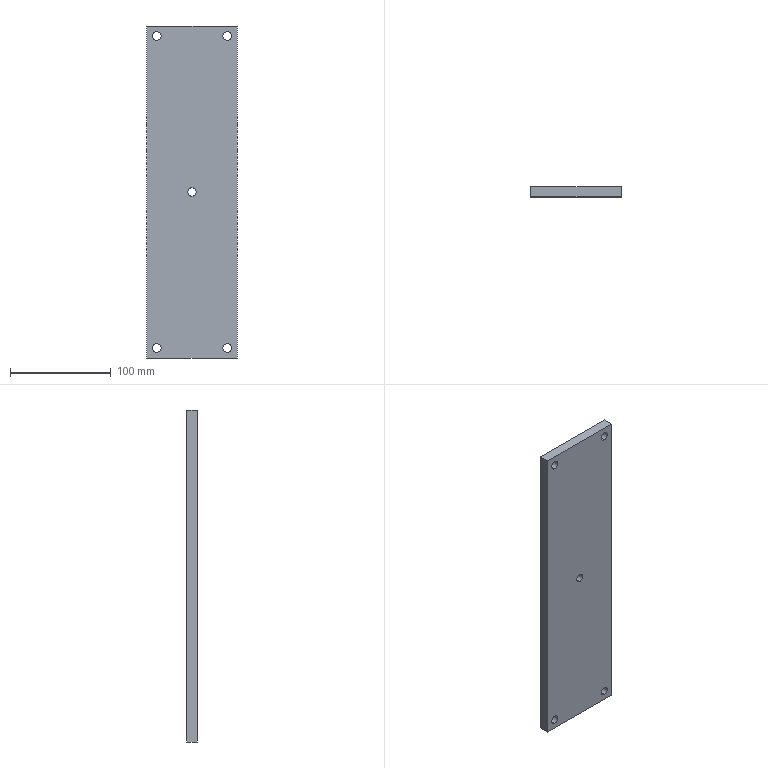Component | SolidWorks | SL021-102-4100.SL4PRT-1 | 1 solid | 16 faces | box 90 x 10 x 330 mm | volume 294163 mm3 | cylinder 10 | plane 6 | commonest cylinder face diameters 8.5 x10 | material AL6061
build123d program:
from build123d import *

# Parameters (mm, degrees)
SKETCH1_W                  = 330
SKETCH1_H                  = 90
BOSS_EXTRUDE1_DEPTH        = 5
F_8_5_8_5_DIAMETER_HOLE1_D = 8.5


with BuildPart() as part:
    # Sketch1 → Boss-Extrude1 (new, symmetric)
    with BuildSketch(Plane.XY):
        Rectangle(SKETCH1_W, SKETCH1_H)
    extrude(amount=BOSS_EXTRUDE1_DEPTH, both=True)

    # 8.5 _8.5_ Diameter Hole1 (through all)
    with Locations(Plane.XY.offset(5)):
        with Locations((-155, 35), (-155, -35), (155, -35), (155, 35), (0, 0)):
            Hole(F_8_5_8_5_DIAMETER_HOLE1_D / 2)


solid = part.part

# Placed as in the assembly
solid = solid.moved(Location((-91.163, 64.501, -151.378), (90, 0, 90)))
STEP:
#1=COLOUR_RGB('',0.7922,0.8196,0.9333);
#2=FILL_AREA_STYLE_COLOUR('',#1);
#3=FILL_AREA_STYLE('',(#2));
#4=SURFACE_STYLE_FILL_AREA(#3);
#5=SURFACE_SIDE_STYLE('',(#4));
#6=SURFACE_STYLE_USAGE(.BOTH.,#5);
#7=PRESENTATION_STYLE_ASSIGNMENT((#6));
#8=CARTESIAN_POINT('',(-4.967,2.736,-12.229));
#9=VERTEX_POINT('',#8);
#10=CARTESIAN_POINT('',(-4.967,2.736,-11.895));
#11=VERTEX_POINT('',#10);
#12=CARTESIAN_POINT('',(-4.967,2.736,-12.062));
#13=DIRECTION('',(0.,-1.,0.));
#14=DIRECTION('',(0.,0.,1.));
#15=AXIS2_PLACEMENT_3D('',#12,#13,#14);
#16=CIRCLE('',#15,0.1673);
#17=EDGE_CURVE('',#9,#11,#16,.T.);
#18=ORIENTED_EDGE('',*,*,#17,.F.);
#19=CARTESIAN_POINT('',(-4.967,2.343,-12.229));
#20=VERTEX_POINT('',#19);
#21=CARTESIAN_POINT('',(-4.967,2.343,-12.229));
#22=DIRECTION('',(0.,-1.,0.));
#23=VECTOR('',#22,39.37);
#24=LINE('',#21,#23);
#25=EDGE_CURVE('',#9,#20,#24,.T.);
#26=ORIENTED_EDGE('',*,*,#25,.T.);
#27=CARTESIAN_POINT('',(-4.967,2.343,-11.895));
#28=VERTEX_POINT('',#27);
#29=CARTESIAN_POINT('',(-4.967,2.343,-12.062));
#30=DIRECTION('',(0.,-1.,0.));
#31=DIRECTION('',(0.,0.,1.));
#32=AXIS2_PLACEMENT_3D('',#29,#30,#31);
#33=CIRCLE('',#32,0.1673);
#34=EDGE_CURVE('',#20,#28,#33,.T.);
#35=ORIENTED_EDGE('',*,*,#34,.T.);
#36=CARTESIAN_POINT('',(-4.967,2.343,-11.895));
#37=DIRECTION('',(0.,-1.,0.));
#38=VECTOR('',#37,39.37);
#39=LINE('',#36,#38);
#40=EDGE_CURVE('',#11,#28,#39,.T.);
#41=ORIENTED_EDGE('',*,*,#40,.F.);
#42=EDGE_LOOP('',(#18,#26,#35,#41));
#43=FACE_OUTER_BOUND('',#42,.T.);
#44=CARTESIAN_POINT('',(-4.967,2.343,-12.062));
#45=DIRECTION('',(0.,-1.,0.));
#46=DIRECTION('',(0.,0.,1.));
#47=AXIS2_PLACEMENT_3D('',#44,#45,#46);
#48=CYLINDRICAL_SURFACE('',#47,0.1673);
#49=ADVANCED_FACE('',(#43),#48,.F.);
#50=CARTESIAN_POINT('',(-2.211,2.736,-12.229));
#51=VERTEX_POINT('',#50);
#52=CARTESIAN_POINT('',(-2.211,2.736,-11.895));
#53=VERTEX_POINT('',#52);
#54=CARTESIAN_POINT('',(-2.211,2.736,-12.062));
#55=DIRECTION('',(0.,-1.,0.));
#56=DIRECTION('',(0.,0.,1.));
#57=AXIS2_PLACEMENT_3D('',#54,#55,#56);
#58=CIRCLE('',#57,0.1673);
#59=EDGE_CURVE('',#51,#53,#58,.T.);
#60=ORIENTED_EDGE('',*,*,#59,.F.);
#61=CARTESIAN_POINT('',(-2.211,2.343,-12.229));
#62=VERTEX_POINT('',#61);
#63=CARTESIAN_POINT('',(-2.211,2.343,-12.229));
#64=DIRECTION('',(0.,-1.,0.));
#65=VECTOR('',#64,39.37);
#66=LINE('',#63,#65);
#67=EDGE_CURVE('',#51,#62,#66,.T.);
#68=ORIENTED_EDGE('',*,*,#67,.T.);
#69=CARTESIAN_POINT('',(-2.211,2.343,-11.895));
#70=VERTEX_POINT('',#69);
#71=CARTESIAN_POINT('',(-2.211,2.343,-12.062));
#72=DIRECTION('',(0.,-1.,0.));
#73=DIRECTION('',(0.,0.,1.));
#74=AXIS2_PLACEMENT_3D('',#71,#72,#73);
#75=CIRCLE('',#74,0.1673);
#76=EDGE_CURVE('',#62,#70,#75,.T.);
#77=ORIENTED_EDGE('',*,*,#76,.T.);
#78=CARTESIAN_POINT('',(-2.211,2.343,-11.895));
#79=DIRECTION('',(0.,-1.,0.));
#80=VECTOR('',#79,39.37);
#81=LINE('',#78,#80);
#82=EDGE_CURVE('',#53,#70,#81,.T.);
#83=ORIENTED_EDGE('',*,*,#82,.F.);
#84=EDGE_LOOP('',(#60,#68,#77,#83));
#85=FACE_OUTER_BOUND('',#84,.T.);
#86=CARTESIAN_POINT('',(-2.211,2.343,-12.062));
#87=DIRECTION('',(0.,-1.,0.));
#88=DIRECTION('',(0.,0.,1.));
#89=AXIS2_PLACEMENT_3D('',#86,#87,#88);
#90=CYLINDRICAL_SURFACE('',#89,0.1673);
#91=ADVANCED_FACE('',(#85),#90,.F.);
#92=CARTESIAN_POINT('',(-2.211,2.736,-0.02474));
#93=VERTEX_POINT('',#92);
#94=CARTESIAN_POINT('',(-2.211,2.736,0.3099));
#95=VERTEX_POINT('',#94);
#96=CARTESIAN_POINT('',(-2.211,2.736,0.1426));
#97=DIRECTION('',(0.,-1.,0.));
#98=DIRECTION('',(0.,0.,1.));
#99=AXIS2_PLACEMENT_3D('',#96,#97,#98);
#100=CIRCLE('',#99,0.1673);
#101=EDGE_CURVE('',#93,#95,#100,.T.);
#102=ORIENTED_EDGE('',*,*,#101,.F.);
#103=CARTESIAN_POINT('',(-2.211,2.343,-0.02474));
#104=VERTEX_POINT('',#103);
#105=CARTESIAN_POINT('',(-2.211,2.343,-0.02474));
#106=DIRECTION('',(0.,-1.,0.));
#107=VECTOR('',#106,39.37);
#108=LINE('',#105,#107);
#109=EDGE_CURVE('',#93,#104,#108,.T.);
#110=ORIENTED_EDGE('',*,*,#109,.T.);
#111=CARTESIAN_POINT('',(-2.211,2.343,0.3099));
#112=VERTEX_POINT('',#111);
#113=CARTESIAN_POINT('',(-2.211,2.343,0.1426));
#114=DIRECTION('',(0.,-1.,0.));
#115=DIRECTION('',(0.,0.,1.));
#116=AXIS2_PLACEMENT_3D('',#113,#114,#115);
#117=CIRCLE('',#116,0.1673);
#118=EDGE_CURVE('',#104,#112,#117,.T.);
#119=ORIENTED_EDGE('',*,*,#118,.T.);
#120=CARTESIAN_POINT('',(-2.211,2.343,0.3099));
#121=DIRECTION('',(0.,-1.,0.));
#122=VECTOR('',#121,39.37);
#123=LINE('',#120,#122);
#124=EDGE_CURVE('',#95,#112,#123,.T.);
#125=ORIENTED_EDGE('',*,*,#124,.F.);
#126=EDGE_LOOP('',(#102,#110,#119,#125));
#127=FACE_OUTER_BOUND('',#126,.T.);
#128=CARTESIAN_POINT('',(-2.211,2.343,0.1426));
#129=DIRECTION('',(0.,-1.,0.));
#130=DIRECTION('',(0.,0.,1.));
#131=AXIS2_PLACEMENT_3D('',#128,#129,#130);
#132=CYLINDRICAL_SURFACE('',#131,0.1673);
#133=ADVANCED_FACE('',(#127),#132,.F.);
#134=CARTESIAN_POINT('',(-4.967,2.736,-0.02474));
#135=VERTEX_POINT('',#134);
#136=CARTESIAN_POINT('',(-4.967,2.736,0.3099));
#137=VERTEX_POINT('',#136);
#138=CARTESIAN_POINT('',(-4.967,2.736,0.1426));
#139=DIRECTION('',(0.,-1.,0.));
#140=DIRECTION('',(0.,0.,1.));
#141=AXIS2_PLACEMENT_3D('',#138,#139,#140);
#142=CIRCLE('',#141,0.1673);
#143=EDGE_CURVE('',#135,#137,#142,.T.);
#144=ORIENTED_EDGE('',*,*,#143,.F.);
#145=CARTESIAN_POINT('',(-4.967,2.343,-0.02474));
#146=VERTEX_POINT('',#145);
#147=CARTESIAN_POINT('',(-4.967,2.343,-0.02474));
#148=DIRECTION('',(0.,-1.,0.));
#149=VECTOR('',#148,39.37);
#150=LINE('',#147,#149);
#151=EDGE_CURVE('',#135,#146,#150,.T.);
#152=ORIENTED_EDGE('',*,*,#151,.T.);
#153=CARTESIAN_POINT('',(-4.967,2.343,0.3099));
#154=VERTEX_POINT('',#153);
#155=CARTESIAN_POINT('',(-4.967,2.343,0.1426));
#156=DIRECTION('',(0.,-1.,0.));
#157=DIRECTION('',(0.,0.,1.));
#158=AXIS2_PLACEMENT_3D('',#155,#156,#157);
#159=CIRCLE('',#158,0.1673);
#160=EDGE_CURVE('',#146,#154,#159,.T.);
#161=ORIENTED_EDGE('',*,*,#160,.T.);
#162=CARTESIAN_POINT('',(-4.967,2.343,0.3099));
#163=DIRECTION('',(0.,-1.,0.));
#164=VECTOR('',#163,39.37);
#165=LINE('',#162,#164);
#166=EDGE_CURVE('',#137,#154,#165,.T.);
#167=ORIENTED_EDGE('',*,*,#166,.F.);
#168=EDGE_LOOP('',(#144,#152,#161,#167));
#169=FACE_OUTER_BOUND('',#168,.T.);
#170=CARTESIAN_POINT('',(-4.967,2.343,0.1426));
#171=DIRECTION('',(0.,-1.,0.));
#172=DIRECTION('',(0.,0.,1.));
#173=AXIS2_PLACEMENT_3D('',#170,#171,#172);
#174=CYLINDRICAL_SURFACE('',#173,0.1673);
#175=ADVANCED_FACE('',(#169),#174,.F.);
#176=CARTESIAN_POINT('',(-3.589,2.736,-6.127));
#177=VERTEX_POINT('',#176);
#178=CARTESIAN_POINT('',(-3.589,2.736,-5.792));
#179=VERTEX_POINT('',#178);
#180=CARTESIAN_POINT('',(-3.589,2.736,-5.96));
#181=DIRECTION('',(0.,-1.,0.));
#182=DIRECTION('',(0.,0.,1.));
#183=AXIS2_PLACEMENT_3D('',#180,#181,#182);
#184=CIRCLE('',#183,0.1673);
#185=EDGE_CURVE('',#177,#179,#184,.T.);
#186=ORIENTED_EDGE('',*,*,#185,.F.);
#187=CARTESIAN_POINT('',(-3.589,2.343,-6.127));
#188=VERTEX_POINT('',#187);
#189=CARTESIAN_POINT('',(-3.589,2.343,-6.127));
#190=DIRECTION('',(0.,-1.,0.));
#191=VECTOR('',#190,39.37);
#192=LINE('',#189,#191);
#193=EDGE_CURVE('',#177,#188,#192,.T.);
#194=ORIENTED_EDGE('',*,*,#193,.T.);
#195=CARTESIAN_POINT('',(-3.589,2.343,-5.792));
#196=VERTEX_POINT('',#195);
#197=CARTESIAN_POINT('',(-3.589,2.343,-5.96));
#198=DIRECTION('',(0.,-1.,0.));
#199=DIRECTION('',(0.,0.,1.));
#200=AXIS2_PLACEMENT_3D('',#197,#198,#199);
#201=CIRCLE('',#200,0.1673);
#202=EDGE_CURVE('',#188,#196,#201,.T.);
#203=ORIENTED_EDGE('',*,*,#202,.T.);
#204=CARTESIAN_POINT('',(-3.589,2.343,-5.792));
#205=DIRECTION('',(0.,-1.,0.));
#206=VECTOR('',#205,39.37);
#207=LINE('',#204,#206);
#208=EDGE_CURVE('',#179,#196,#207,.T.);
#209=ORIENTED_EDGE('',*,*,#208,.F.);
#210=EDGE_LOOP('',(#186,#194,#203,#209));
#211=FACE_OUTER_BOUND('',#210,.T.);
#212=CARTESIAN_POINT('',(-3.589,2.343,-5.96));
#213=DIRECTION('',(0.,-1.,0.));
#214=DIRECTION('',(0.,0.,1.));
#215=AXIS2_PLACEMENT_3D('',#212,#213,#214);
#216=CYLINDRICAL_SURFACE('',#215,0.1673);
#217=ADVANCED_FACE('',(#211),#216,.F.);
#218=CARTESIAN_POINT('',(-1.817,2.736,0.5363));
#219=VERTEX_POINT('',#218);
#220=CARTESIAN_POINT('',(-5.361,2.736,0.5363));
#221=VERTEX_POINT('',#220);
#222=CARTESIAN_POINT('',(-1.817,2.736,0.5363));
#223=DIRECTION('',(-1.,-0.,-0.));
#224=VECTOR('',#223,39.37);
#225=LINE('',#222,#224);
#226=EDGE_CURVE('',#219,#221,#225,.T.);
#227=ORIENTED_EDGE('',*,*,#226,.T.);
#228=CARTESIAN_POINT('',(-5.361,2.343,0.5363));
#229=VERTEX_POINT('',#228);
#230=CARTESIAN_POINT('',(-5.361,2.343,0.5363));
#231=DIRECTION('',(-0.,1.,-0.));
#232=VECTOR('',#231,39.37);
#233=LINE('',#230,#232);
#234=EDGE_CURVE('',#229,#221,#233,.T.);
#235=ORIENTED_EDGE('',*,*,#234,.F.);
#236=CARTESIAN_POINT('',(-1.817,2.343,0.5363));
#237=VERTEX_POINT('',#236);
#238=CARTESIAN_POINT('',(-1.817,2.343,0.5363));
#239=DIRECTION('',(-1.,-0.,-0.));
#240=VECTOR('',#239,39.37);
#241=LINE('',#238,#240);
#242=EDGE_CURVE('',#237,#229,#241,.T.);
#243=ORIENTED_EDGE('',*,*,#242,.F.);
#244=CARTESIAN_POINT('',(-1.817,2.343,0.5363));
#245=DIRECTION('',(-0.,1.,-0.));
#246=VECTOR('',#245,39.37);
#247=LINE('',#244,#246);
#248=EDGE_CURVE('',#237,#219,#247,.T.);
#249=ORIENTED_EDGE('',*,*,#248,.T.);
#250=EDGE_LOOP('',(#227,#235,#243,#249));
#251=FACE_OUTER_BOUND('',#250,.T.);
#252=CARTESIAN_POINT('',(-1.817,2.343,0.5363));
#253=DIRECTION('',(0.,-0.,-1.));
#254=DIRECTION('',(0.,-1.,0.));
#255=AXIS2_PLACEMENT_3D('',#252,#253,#254);
#256=PLANE('',#255);
#257=ADVANCED_FACE('',(#251),#256,.F.);
#258=CARTESIAN_POINT('',(-5.361,2.736,-12.456));
#259=VERTEX_POINT('',#258);
#260=CARTESIAN_POINT('',(-5.361,2.736,-12.456));
#261=DIRECTION('',(0.,-0.,-1.));
#262=VECTOR('',#261,39.37);
#263=LINE('',#260,#262);
#264=EDGE_CURVE('',#221,#259,#263,.T.);
#265=ORIENTED_EDGE('',*,*,#264,.T.);
#266=CARTESIAN_POINT('',(-5.361,2.343,-12.456));
#267=VERTEX_POINT('',#266);
#268=CARTESIAN_POINT('',(-5.361,2.343,-12.456));
#269=DIRECTION('',(-0.,1.,-0.));
#270=VECTOR('',#269,39.37);
#271=LINE('',#268,#270);
#272=EDGE_CURVE('',#267,#259,#271,.T.);
#273=ORIENTED_EDGE('',*,*,#272,.F.);
#274=CARTESIAN_POINT('',(-5.361,2.343,-12.456));
#275=DIRECTION('',(0.,-0.,-1.));
#276=VECTOR('',#275,39.37);
#277=LINE('',#274,#276);
#278=EDGE_CURVE('',#229,#267,#277,.T.);
#279=ORIENTED_EDGE('',*,*,#278,.F.);
#280=ORIENTED_EDGE('',*,*,#234,.T.);
#281=EDGE_LOOP('',(#265,#273,#279,#280));
#282=FACE_OUTER_BOUND('',#281,.T.);
#283=CARTESIAN_POINT('',(-5.361,2.343,-12.456));
#284=DIRECTION('',(1.,0.,0.));
#285=DIRECTION('',(-0.,1.,-0.));
#286=AXIS2_PLACEMENT_3D('',#283,#284,#285);
#287=PLANE('',#286);
#288=ADVANCED_FACE('',(#282),#287,.F.);
#289=CARTESIAN_POINT('',(-1.817,2.736,-12.456));
#290=VERTEX_POINT('',#289);
#291=CARTESIAN_POINT('',(-1.817,2.736,-12.456));
#292=DIRECTION('',(1.,0.,0.));
#293=VECTOR('',#292,39.37);
#294=LINE('',#291,#293);
#295=EDGE_CURVE('',#259,#290,#294,.T.);
#296=ORIENTED_EDGE('',*,*,#295,.T.);
#297=CARTESIAN_POINT('',(-1.817,2.343,-12.456));
#298=VERTEX_POINT('',#297);
#299=CARTESIAN_POINT('',(-1.817,2.343,-12.456));
#300=DIRECTION('',(-0.,1.,-0.));
#301=VECTOR('',#300,39.37);
#302=LINE('',#299,#301);
#303=EDGE_CURVE('',#298,#290,#302,.T.);
#304=ORIENTED_EDGE('',*,*,#303,.F.);
#305=CARTESIAN_POINT('',(-1.817,2.343,-12.456));
#306=DIRECTION('',(1.,0.,0.));
#307=VECTOR('',#306,39.37);
#308=LINE('',#305,#307);
#309=EDGE_CURVE('',#267,#298,#308,.T.);
#310=ORIENTED_EDGE('',*,*,#309,.F.);
#311=ORIENTED_EDGE('',*,*,#272,.T.);
#312=EDGE_LOOP('',(#296,#304,#310,#311));
#313=FACE_OUTER_BOUND('',#312,.T.);
#314=CARTESIAN_POINT('',(-1.817,2.343,-12.456));
#315=DIRECTION('',(-0.,0.,1.));
#316=DIRECTION('',(-0.,1.,-0.));
#317=AXIS2_PLACEMENT_3D('',#314,#315,#316);
#318=PLANE('',#317);
#319=ADVANCED_FACE('',(#313),#318,.F.);
#320=CARTESIAN_POINT('',(-1.817,2.736,-12.456));
#321=DIRECTION('',(-0.,0.,1.));
#322=VECTOR('',#321,39.37);
#323=LINE('',#320,#322);
#324=EDGE_CURVE('',#290,#219,#323,.T.);
#325=ORIENTED_EDGE('',*,*,#324,.T.);
#326=ORIENTED_EDGE('',*,*,#248,.F.);
#327=CARTESIAN_POINT('',(-1.817,2.343,-12.456));
#328=DIRECTION('',(-0.,0.,1.));
#329=VECTOR('',#328,39.37);
#330=LINE('',#327,#329);
#331=EDGE_CURVE('',#298,#237,#330,.T.);
#332=ORIENTED_EDGE('',*,*,#331,.F.);
#333=ORIENTED_EDGE('',*,*,#303,.T.);
#334=EDGE_LOOP('',(#325,#326,#332,#333));
#335=FACE_OUTER_BOUND('',#334,.T.);
#336=CARTESIAN_POINT('',(-1.817,2.343,-12.456));
#337=DIRECTION('',(-1.,-0.,-0.));
#338=DIRECTION('',(0.,-1.,0.));
#339=AXIS2_PLACEMENT_3D('',#336,#337,#338);
#340=PLANE('',#339);
#341=ADVANCED_FACE('',(#335),#340,.F.);
#342=CARTESIAN_POINT('',(-4.967,2.343,-12.062));
#343=DIRECTION('',(0.,-1.,0.));
#344=DIRECTION('',(0.,0.,1.));
#345=AXIS2_PLACEMENT_3D('',#342,#343,#344);
#346=CIRCLE('',#345,0.1673);
#347=EDGE_CURVE('',#28,#20,#346,.T.);
#348=ORIENTED_EDGE('',*,*,#347,.F.);
#349=ORIENTED_EDGE('',*,*,#34,.F.);
#350=EDGE_LOOP('',(#348,#349));
#351=FACE_BOUND('',#350,.T.);
#352=CARTESIAN_POINT('',(-2.211,2.343,-12.062));
#353=DIRECTION('',(0.,-1.,0.));
#354=DIRECTION('',(0.,0.,1.));
#355=AXIS2_PLACEMENT_3D('',#352,#353,#354);
#356=CIRCLE('',#355,0.1673);
#357=EDGE_CURVE('',#70,#62,#356,.T.);
#358=ORIENTED_EDGE('',*,*,#357,.F.);
#359=ORIENTED_EDGE('',*,*,#76,.F.);
#360=EDGE_LOOP('',(#358,#359));
#361=FACE_BOUND('',#360,.T.);
#362=CARTESIAN_POINT('',(-2.211,2.343,0.1426));
#363=DIRECTION('',(0.,-1.,0.));
#364=DIRECTION('',(0.,0.,1.));
#365=AXIS2_PLACEMENT_3D('',#362,#363,#364);
#366=CIRCLE('',#365,0.1673);
#367=EDGE_CURVE('',#112,#104,#366,.T.);
#368=ORIENTED_EDGE('',*,*,#367,.F.);
#369=ORIENTED_EDGE('',*,*,#118,.F.);
#370=EDGE_LOOP('',(#368,#369));
#371=FACE_BOUND('',#370,.T.);
#372=CARTESIAN_POINT('',(-4.967,2.343,0.1426));
#373=DIRECTION('',(0.,-1.,0.));
#374=DIRECTION('',(0.,0.,1.));
#375=AXIS2_PLACEMENT_3D('',#372,#373,#374);
#376=CIRCLE('',#375,0.1673);
#377=EDGE_CURVE('',#154,#146,#376,.T.);
#378=ORIENTED_EDGE('',*,*,#377,.F.);
#379=ORIENTED_EDGE('',*,*,#160,.F.);
#380=EDGE_LOOP('',(#378,#379));
#381=FACE_BOUND('',#380,.T.);
#382=CARTESIAN_POINT('',(-3.589,2.343,-5.96));
#383=DIRECTION('',(0.,-1.,0.));
#384=DIRECTION('',(0.,0.,1.));
#385=AXIS2_PLACEMENT_3D('',#382,#383,#384);
#386=CIRCLE('',#385,0.1673);
#387=EDGE_CURVE('',#196,#188,#386,.T.);
#388=ORIENTED_EDGE('',*,*,#387,.F.);
#389=ORIENTED_EDGE('',*,*,#202,.F.);
#390=EDGE_LOOP('',(#388,#389));
#391=FACE_BOUND('',#390,.T.);
#392=ORIENTED_EDGE('',*,*,#242,.T.);
#393=ORIENTED_EDGE('',*,*,#278,.T.);
#394=ORIENTED_EDGE('',*,*,#309,.T.);
#395=ORIENTED_EDGE('',*,*,#331,.T.);
#396=EDGE_LOOP('',(#392,#393,#394,#395));
#397=FACE_OUTER_BOUND('',#396,.T.);
#398=CARTESIAN_POINT('',(-3.589,2.343,-5.96));
#399=DIRECTION('',(-0.,1.,-0.));
#400=DIRECTION('',(0.,-0.,-1.));
#401=AXIS2_PLACEMENT_3D('',#398,#399,#400);
#402=PLANE('',#401);
#403=ADVANCED_FACE('',(#351,#361,#371,#381,#391,#397),#402,.F.);
#404=CARTESIAN_POINT('',(-4.967,2.736,-12.062));
#405=DIRECTION('',(0.,-1.,0.));
#406=DIRECTION('',(0.,0.,1.));
#407=AXIS2_PLACEMENT_3D('',#404,#405,#406);
#408=CIRCLE('',#407,0.1673);
#409=EDGE_CURVE('',#11,#9,#408,.T.);
#410=ORIENTED_EDGE('',*,*,#409,.T.);
#411=ORIENTED_EDGE('',*,*,#17,.T.);
#412=EDGE_LOOP('',(#410,#411));
#413=FACE_BOUND('',#412,.T.);
#414=CARTESIAN_POINT('',(-2.211,2.736,-12.062));
#415=DIRECTION('',(0.,-1.,0.));
#416=DIRECTION('',(0.,0.,1.));
#417=AXIS2_PLACEMENT_3D('',#414,#415,#416);
#418=CIRCLE('',#417,0.1673);
#419=EDGE_CURVE('',#53,#51,#418,.T.);
#420=ORIENTED_EDGE('',*,*,#419,.T.);
#421=ORIENTED_EDGE('',*,*,#59,.T.);
#422=EDGE_LOOP('',(#420,#421));
#423=FACE_BOUND('',#422,.T.);
#424=CARTESIAN_POINT('',(-2.211,2.736,0.1426));
#425=DIRECTION('',(0.,-1.,0.));
#426=DIRECTION('',(0.,0.,1.));
#427=AXIS2_PLACEMENT_3D('',#424,#425,#426);
#428=CIRCLE('',#427,0.1673);
#429=EDGE_CURVE('',#95,#93,#428,.T.);
#430=ORIENTED_EDGE('',*,*,#429,.T.);
#431=ORIENTED_EDGE('',*,*,#101,.T.);
#432=EDGE_LOOP('',(#430,#431));
#433=FACE_BOUND('',#432,.T.);
#434=CARTESIAN_POINT('',(-4.967,2.736,0.1426));
#435=DIRECTION('',(0.,-1.,0.));
#436=DIRECTION('',(0.,0.,1.));
#437=AXIS2_PLACEMENT_3D('',#434,#435,#436);
#438=CIRCLE('',#437,0.1673);
#439=EDGE_CURVE('',#137,#135,#438,.T.);
#440=ORIENTED_EDGE('',*,*,#439,.T.);
#441=ORIENTED_EDGE('',*,*,#143,.T.);
#442=EDGE_LOOP('',(#440,#441));
#443=FACE_BOUND('',#442,.T.);
#444=CARTESIAN_POINT('',(-3.589,2.736,-5.96));
#445=DIRECTION('',(0.,-1.,0.));
#446=DIRECTION('',(0.,0.,1.));
#447=AXIS2_PLACEMENT_3D('',#444,#445,#446);
#448=CIRCLE('',#447,0.1673);
#449=EDGE_CURVE('',#179,#177,#448,.T.);
#450=ORIENTED_EDGE('',*,*,#449,.T.);
#451=ORIENTED_EDGE('',*,*,#185,.T.);
#452=EDGE_LOOP('',(#450,#451));
#453=FACE_BOUND('',#452,.T.);
#454=ORIENTED_EDGE('',*,*,#226,.F.);
#455=ORIENTED_EDGE('',*,*,#324,.F.);
#456=ORIENTED_EDGE('',*,*,#295,.F.);
#457=ORIENTED_EDGE('',*,*,#264,.F.);
#458=EDGE_LOOP('',(#454,#455,#456,#457));
#459=FACE_OUTER_BOUND('',#458,.T.);
#460=CARTESIAN_POINT('',(-3.589,2.736,-5.96));
#461=DIRECTION('',(-0.,1.,-0.));
#462=DIRECTION('',(0.,-0.,-1.));
#463=AXIS2_PLACEMENT_3D('',#460,#461,#462);
#464=PLANE('',#463);
#465=ADVANCED_FACE('',(#413,#423,#433,#443,#453,#459),#464,.T.);
#466=ORIENTED_EDGE('',*,*,#193,.F.);
#467=ORIENTED_EDGE('',*,*,#449,.F.);
#468=ORIENTED_EDGE('',*,*,#208,.T.);
#469=ORIENTED_EDGE('',*,*,#387,.T.);
#470=EDGE_LOOP('',(#466,#467,#468,#469));
#471=FACE_OUTER_BOUND('',#470,.T.);
#472=CARTESIAN_POINT('',(-3.589,2.343,-5.96));
#473=DIRECTION('',(0.,-1.,0.));
#474=DIRECTION('',(0.,0.,1.));
#475=AXIS2_PLACEMENT_3D('',#472,#473,#474);
#476=CYLINDRICAL_SURFACE('',#475,0.1673);
#477=ADVANCED_FACE('',(#471),#476,.F.);
#478=ORIENTED_EDGE('',*,*,#151,.F.);
#479=ORIENTED_EDGE('',*,*,#439,.F.);
#480=ORIENTED_EDGE('',*,*,#166,.T.);
#481=ORIENTED_EDGE('',*,*,#377,.T.);
#482=EDGE_LOOP('',(#478,#479,#480,#481));
#483=FACE_OUTER_BOUND('',#482,.T.);
#484=CARTESIAN_POINT('',(-4.967,2.343,0.1426));
#485=DIRECTION('',(0.,-1.,0.));
#486=DIRECTION('',(0.,0.,1.));
#487=AXIS2_PLACEMENT_3D('',#484,#485,#486);
#488=CYLINDRICAL_SURFACE('',#487,0.1673);
#489=ADVANCED_FACE('',(#483),#488,.F.);
#490=ORIENTED_EDGE('',*,*,#109,.F.);
#491=ORIENTED_EDGE('',*,*,#429,.F.);
#492=ORIENTED_EDGE('',*,*,#124,.T.);
#493=ORIENTED_EDGE('',*,*,#367,.T.);
#494=EDGE_LOOP('',(#490,#491,#492,#493));
#495=FACE_OUTER_BOUND('',#494,.T.);
#496=CARTESIAN_POINT('',(-2.211,2.343,0.1426));
#497=DIRECTION('',(0.,-1.,0.));
#498=DIRECTION('',(0.,0.,1.));
#499=AXIS2_PLACEMENT_3D('',#496,#497,#498);
#500=CYLINDRICAL_SURFACE('',#499,0.1673);
#501=ADVANCED_FACE('',(#495),#500,.F.);
#502=ORIENTED_EDGE('',*,*,#67,.F.);
#503=ORIENTED_EDGE('',*,*,#419,.F.);
#504=ORIENTED_EDGE('',*,*,#82,.T.);
#505=ORIENTED_EDGE('',*,*,#357,.T.);
#506=EDGE_LOOP('',(#502,#503,#504,#505));
#507=FACE_OUTER_BOUND('',#506,.T.);
#508=CARTESIAN_POINT('',(-2.211,2.343,-12.062));
#509=DIRECTION('',(0.,-1.,0.));
#510=DIRECTION('',(0.,0.,1.));
#511=AXIS2_PLACEMENT_3D('',#508,#509,#510);
#512=CYLINDRICAL_SURFACE('',#511,0.1673);
#513=ADVANCED_FACE('',(#507),#512,.F.);
#514=ORIENTED_EDGE('',*,*,#25,.F.);
#515=ORIENTED_EDGE('',*,*,#409,.F.);
#516=ORIENTED_EDGE('',*,*,#40,.T.);
#517=ORIENTED_EDGE('',*,*,#347,.T.);
#518=EDGE_LOOP('',(#514,#515,#516,#517));
#519=FACE_OUTER_BOUND('',#518,.T.);
#520=CARTESIAN_POINT('',(-4.967,2.343,-12.062));
#521=DIRECTION('',(0.,-1.,0.));
#522=DIRECTION('',(0.,0.,1.));
#523=AXIS2_PLACEMENT_3D('',#520,#521,#522);
#524=CYLINDRICAL_SURFACE('',#523,0.1673);
#525=ADVANCED_FACE('',(#519),#524,.F.);
#526=CLOSED_SHELL('',(#49,#91,#133,#175,#217,#257,#288,#319,#341,#403,#465,#477,#489,#501,#513,#525));
#527=MANIFOLD_SOLID_BREP('',#526);
#528=STYLED_ITEM('',(#7),#527);
#529=(LENGTH_UNIT()NAMED_UNIT(*)SI_UNIT($,.METRE.));
#530=LENGTH_MEASURE_WITH_UNIT(LENGTH_MEASURE(0.0254),#529);
#531=DIMENSIONAL_EXPONENTS(1.,0.,0.,0.,0.,0.,0.);
#532=(CONVERSION_BASED_UNIT('',#530)LENGTH_UNIT()NAMED_UNIT(#531));
#533=UNCERTAINTY_MEASURE_WITH_UNIT(LENGTH_MEASURE(0.00001),#532,'','');
#534=(NAMED_UNIT(*)PLANE_ANGLE_UNIT()SI_UNIT($,.RADIAN.));
#535=(NAMED_UNIT(*)SI_UNIT($,.STERADIAN.)SOLID_ANGLE_UNIT());
#536=(GEOMETRIC_REPRESENTATION_CONTEXT(3)GLOBAL_UNCERTAINTY_ASSIGNED_CONTEXT((#533))GLOBAL_UNIT_ASSIGNED_CONTEXT((#532,#534,#535))REPRESENTATION_CONTEXT('',''));
#537=MECHANICAL_DESIGN_GEOMETRIC_PRESENTATION_REPRESENTATION('',(#528),#536);
#538=CARTESIAN_POINT('',(0.,0.,0.));
#539=DIRECTION('',(0.,0.,1.));
#540=DIRECTION('',(1.,0.,0.));
#541=AXIS2_PLACEMENT_3D('',#538,#539,#540);
#542=(LENGTH_UNIT()NAMED_UNIT(*)SI_UNIT($,.METRE.));
#543=LENGTH_MEASURE_WITH_UNIT(LENGTH_MEASURE(0.0254),#542);
#544=DIMENSIONAL_EXPONENTS(1.,0.,0.,0.,0.,0.,0.);
#545=(CONVERSION_BASED_UNIT('',#543)LENGTH_UNIT()NAMED_UNIT(#544));
#546=UNCERTAINTY_MEASURE_WITH_UNIT(LENGTH_MEASURE(0.00001),#545,'','');
#547=(NAMED_UNIT(*)PLANE_ANGLE_UNIT()SI_UNIT($,.RADIAN.));
#548=(NAMED_UNIT(*)SI_UNIT($,.STERADIAN.)SOLID_ANGLE_UNIT());
#549=(GEOMETRIC_REPRESENTATION_CONTEXT(3)GLOBAL_UNCERTAINTY_ASSIGNED_CONTEXT((#546))GLOBAL_UNIT_ASSIGNED_CONTEXT((#545,#547,#548))REPRESENTATION_CONTEXT('',''));
#550=ADVANCED_BREP_SHAPE_REPRESENTATION('',(#527,#541),#549);
#551=PRESENTATION_LAYER_ASSIGNMENT('','',(#528));